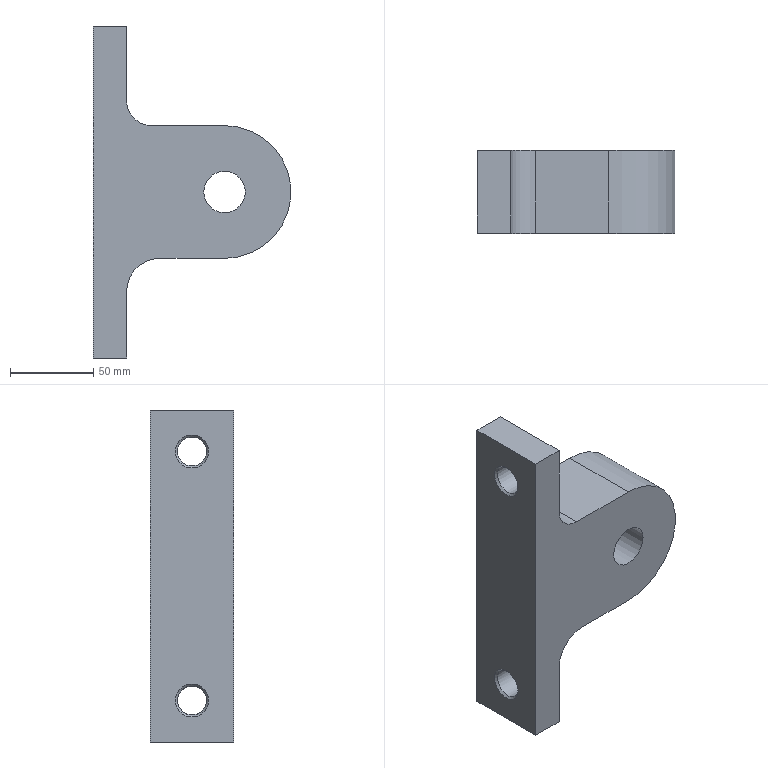Component | NX | LEAD_SCREW_MOUNT | 1 solid | 19 faces | volume 534025 mm3 | plane 9 | cylinder 6 | cone 4 | commonest cylinder face diameters 17.5 x2 40 x1 80 x1 30 x1 25 x1